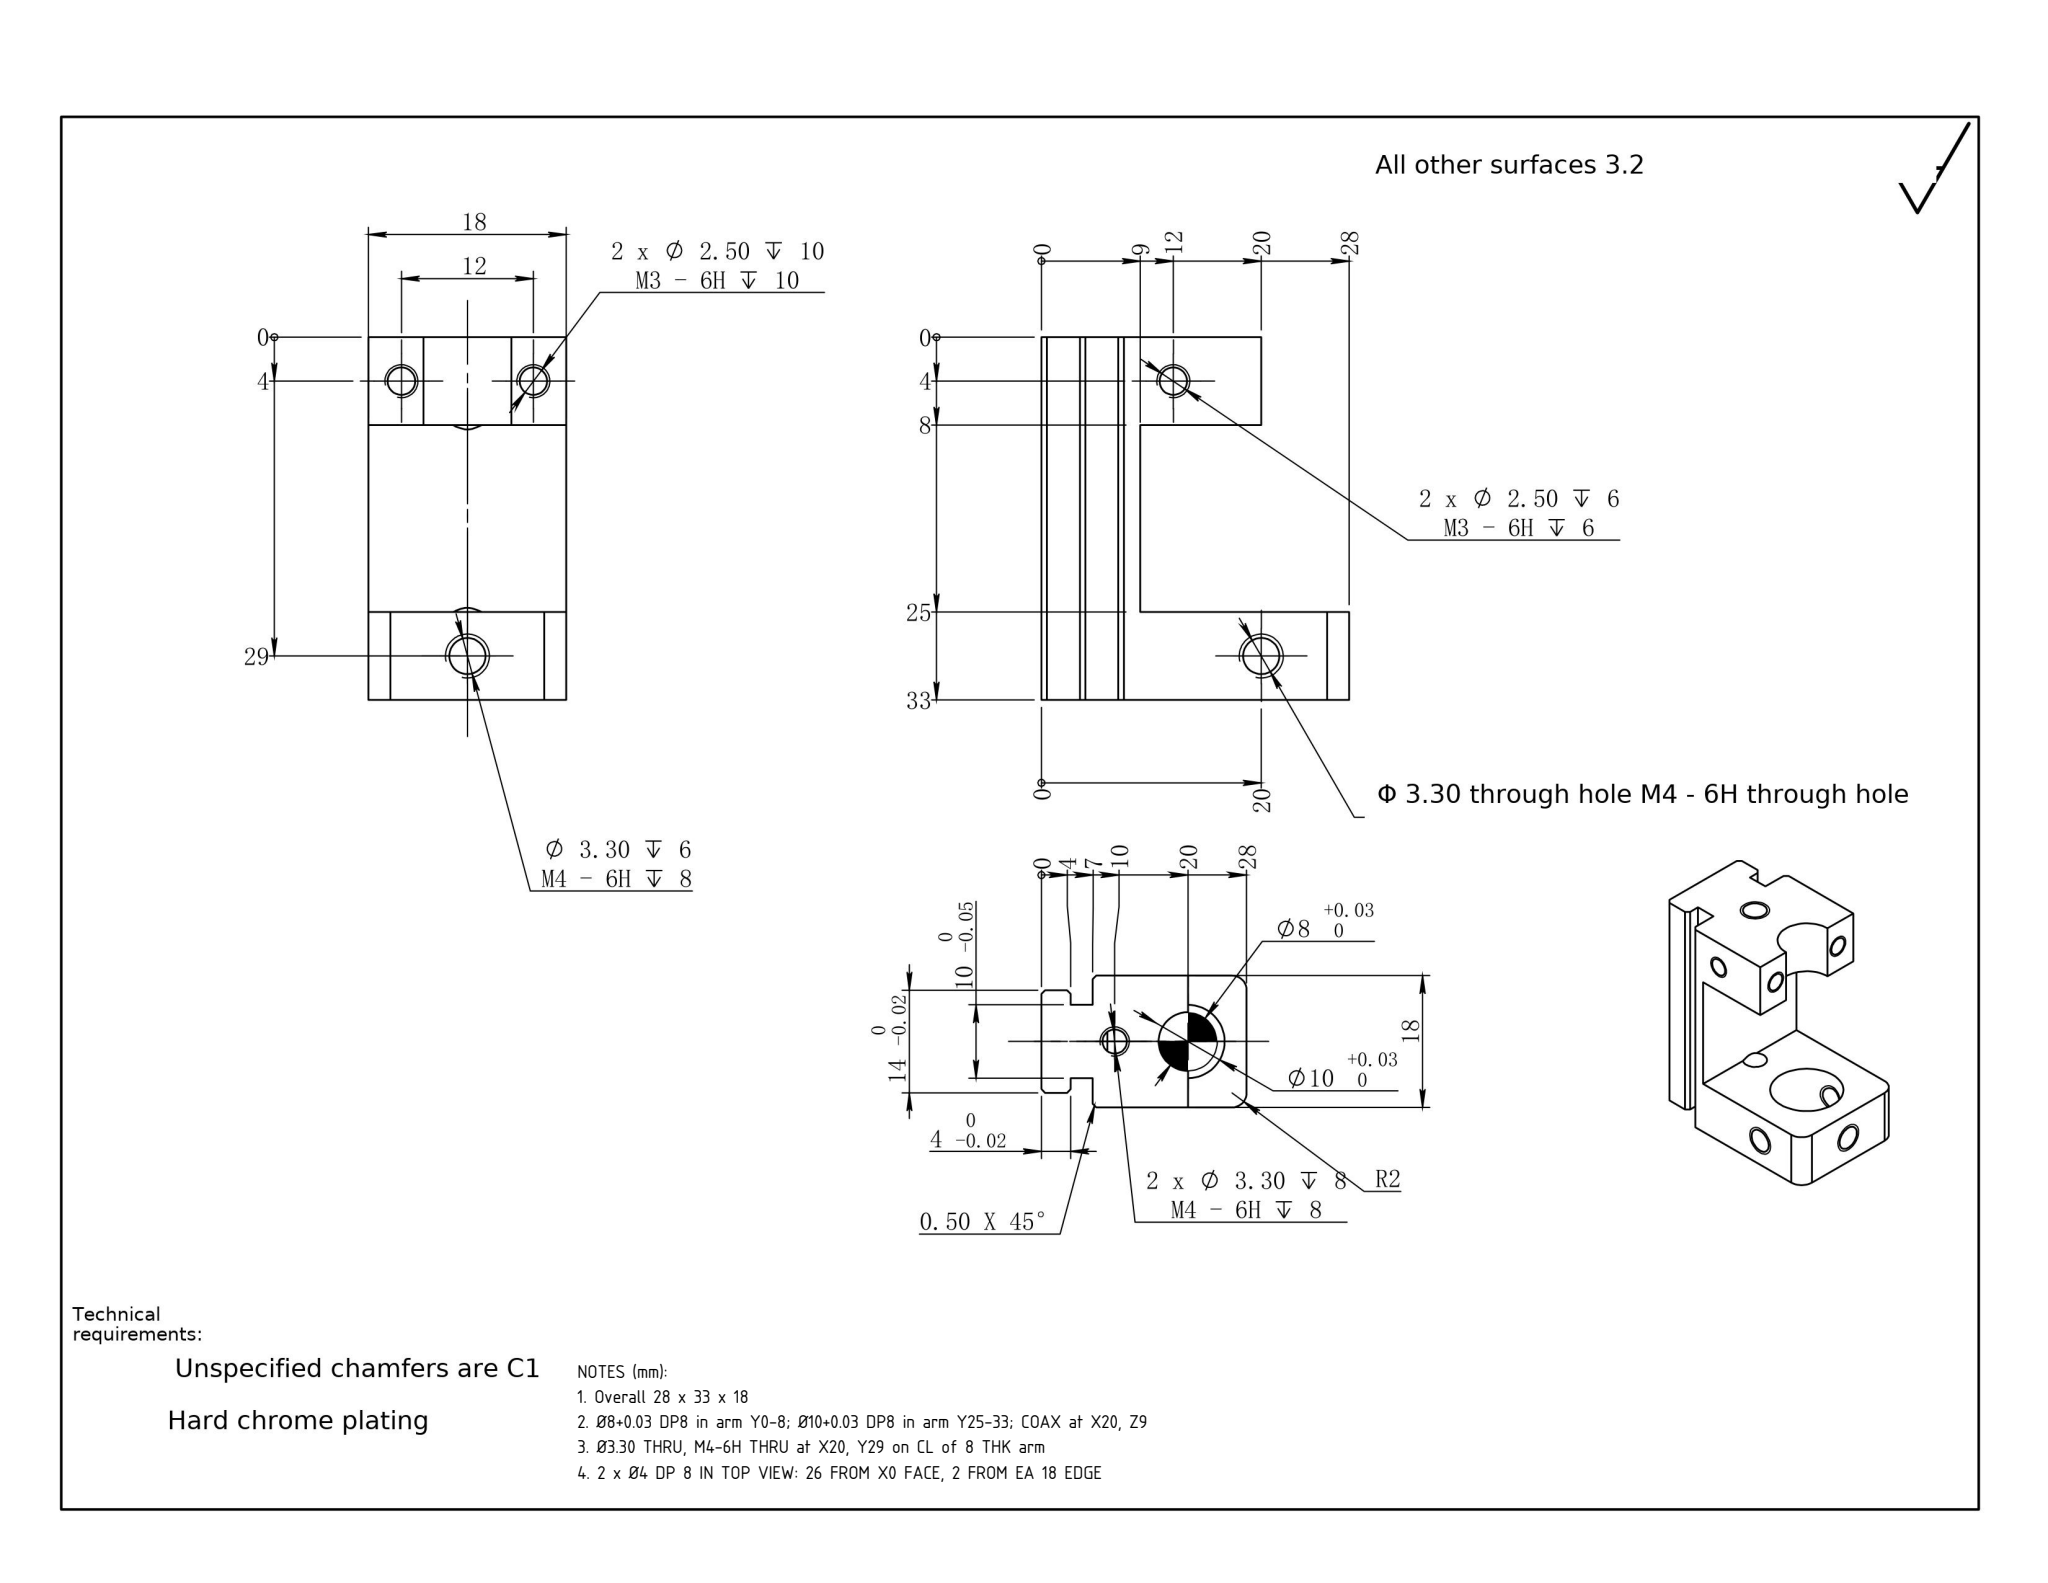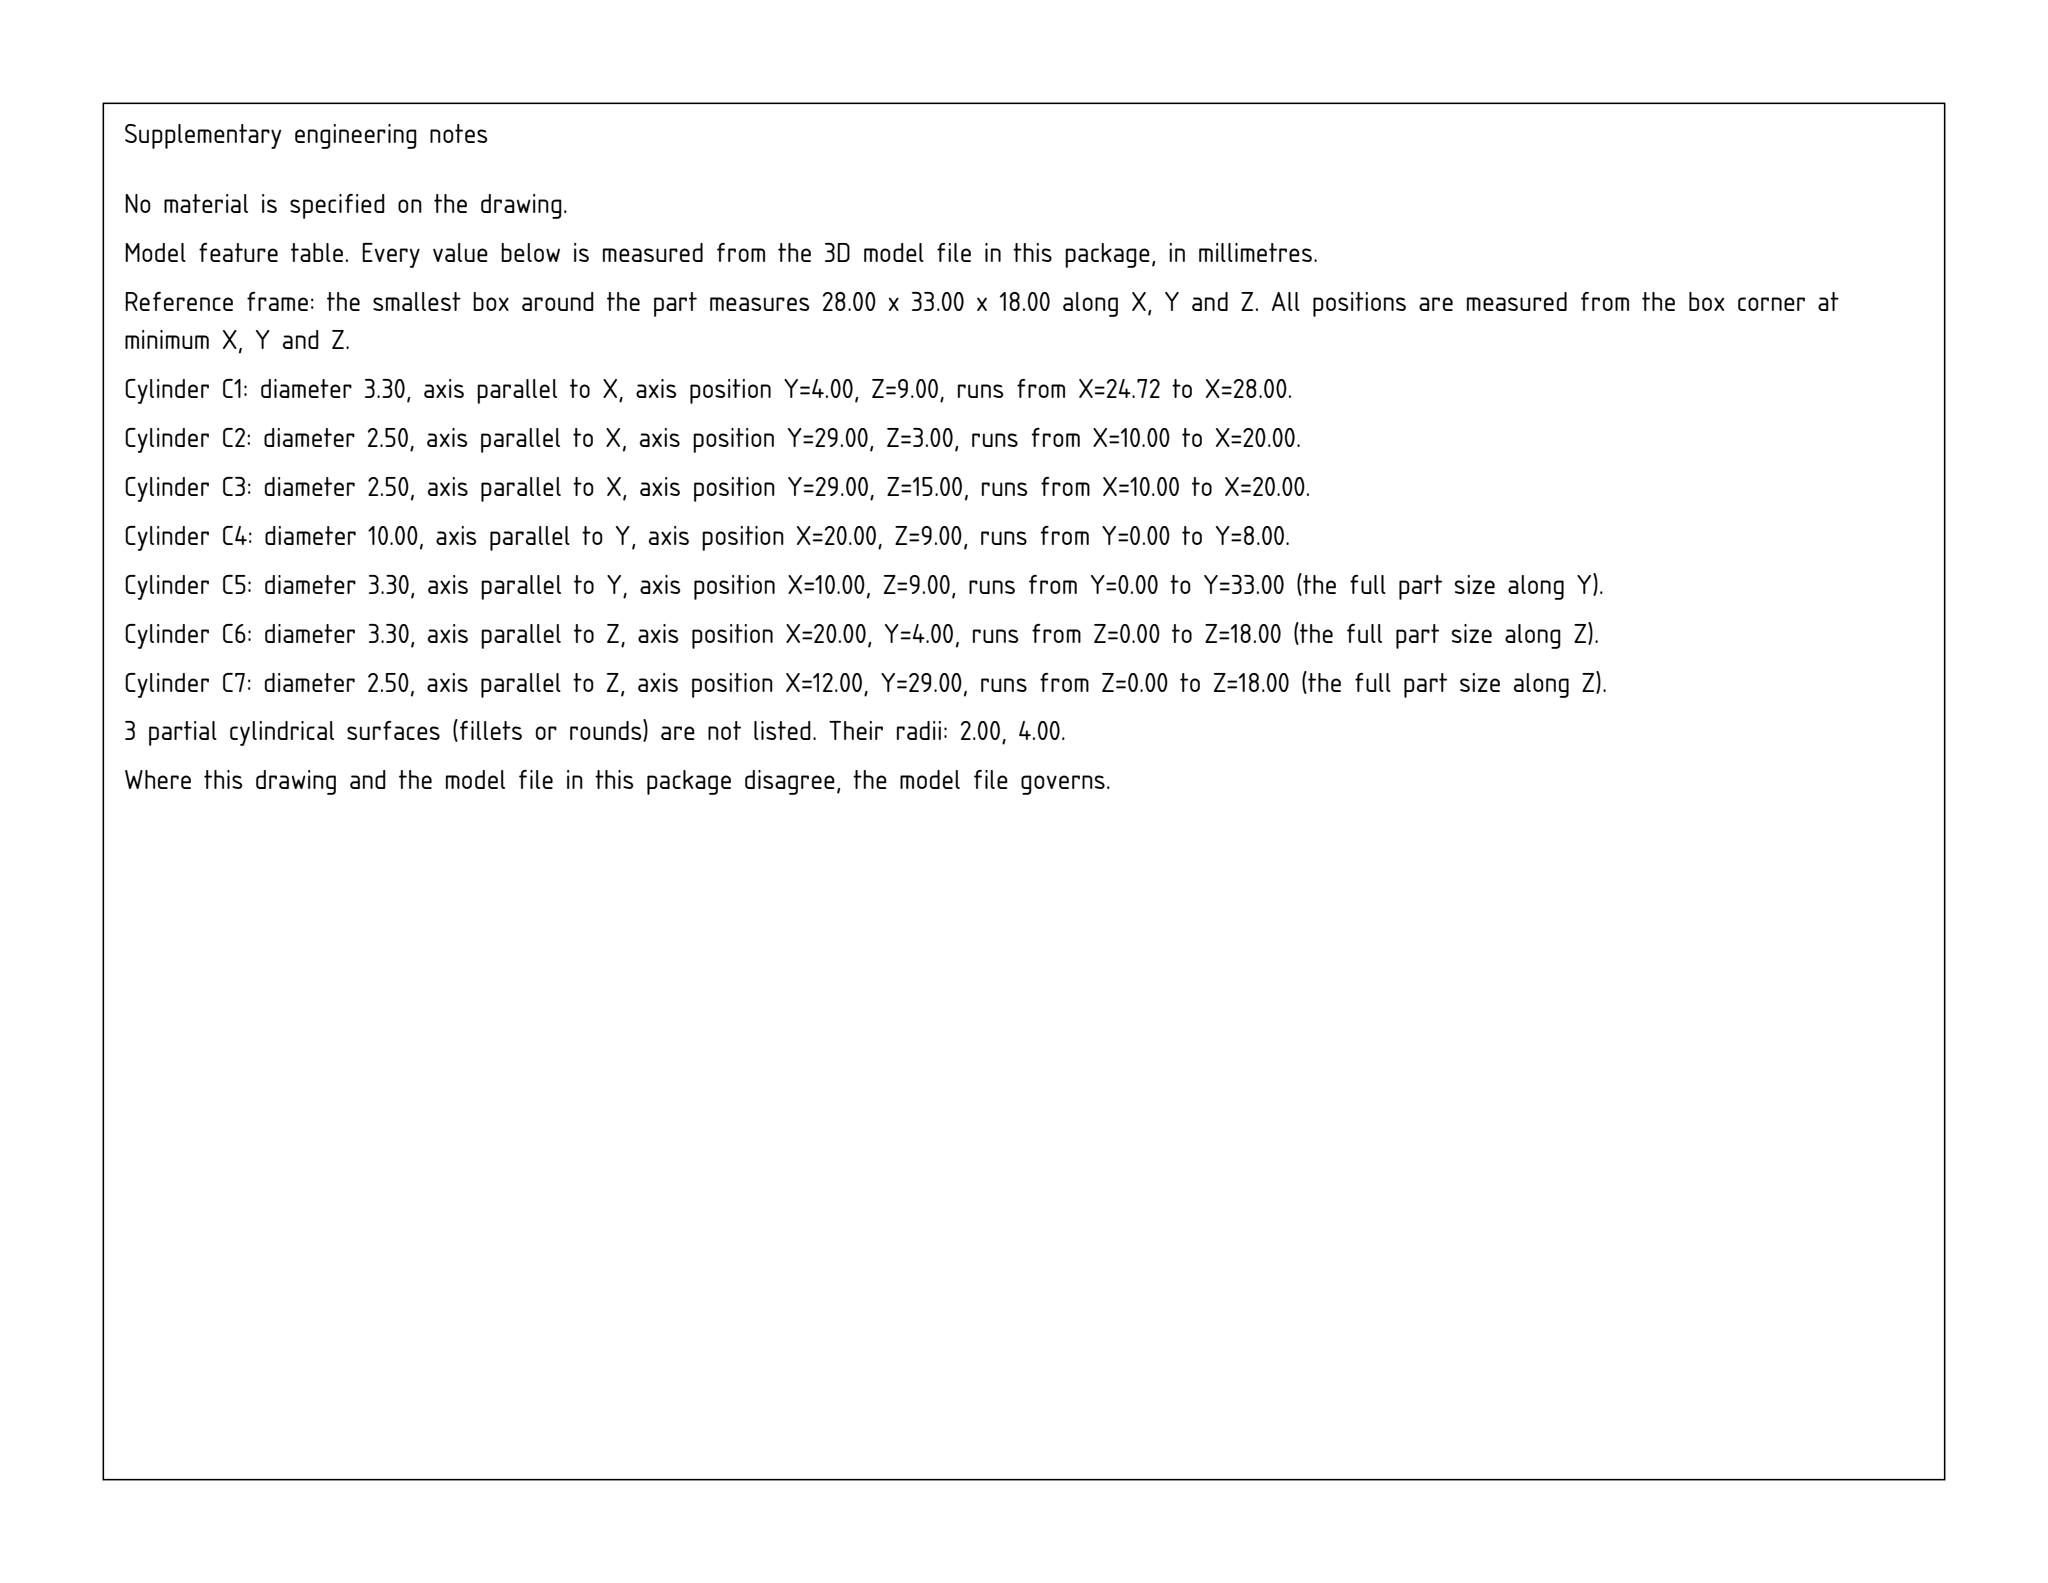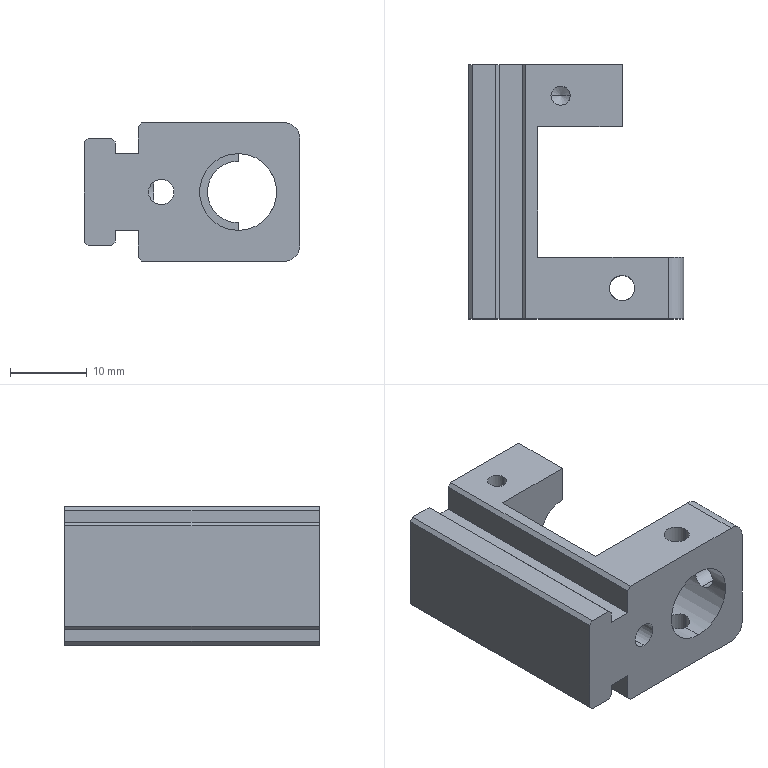Part | SolidWorks | mm | 1 solid | 66 faces | box 28 x 33 x 18 mm | volume 7104 mm3 | cylinder 31 | plane 25 | cone 10 | commonest cylinder face diameters 2.5 x16 3.3 x10 10 x2 4 x2 8 x1
Drawing notes:
Overall 28 x 33 x 18 | from the solid: bbox_xyz [28.001, 33.001, 18.001]
Ø8+0.03 DP8 in arm Y0-8; Ø10+0.03 DP8 in arm Y25-33; COAX at X20, Z9 | from the solid: cylinders [8.0,'y',[20,null,9],8.0] and [10.0,'y',[20,null,9],8.0]; arm faces y0/8 and y25/33 give 8 THK; Ø3.3 x-hole L3.28 and Ø3.3 z-hole L4.28 break into r5 bore, placing Ø10 in the M4-hole arm
Ø3.30 THRU, M4-6H THRU at X20, Y29 on CL of 8 THK arm | from the solid: cylinder [3.3,'z',[20,4(model),null],4.28] = drawing Y 33-4 = 29; arm faces y25/y33
2 x Ø4 DP 8 IN TOP VIEW: 26 FROM X0 FACE, 2 FROM EA 18 EDGE | from the solid: cylinders [4.0,"y",[26.0,null,2.0],8.0] and [4.0,"y",[26.0,null,16.0],8.0]; bbox 28 x 33 x 18, Z planes 0 and 18
build123d program:
from build123d import *

# Parameters (mm, degrees)
SKETCH2_W             = 18
SKETCH2_H             = 33
BOSS_EXTRUDE1_DEPTH   = 28
SKETCH3_W             = 38
SKETCH3_H             = 17
CUT_EXTRUDE1_DEPTH    = 38.152
SKETCH5_R             = 4
CUT_EXTRUDE2_DEPTH    = 45.204
SKETCH6_W             = 3
SKETCH6_H             = 8
CUT_EXTRUDE3_DEPTH    = 45.204
SKETCH14_W            = 4
SKETCH14_H            = 2
CUT_EXTRUDE5_DEPTH    = 45.204
SKETCH10_W            = 16
SKETCH10_H            = 18
CUT_EXTRUDE4_DEPTH    = 10
M3_TAPPED_HOLE1_D     = 2.5
M3_TAPPED_HOLE1_DEPTH = 10
M3_TAPPED_HOLE1_TIP   = 0.7511
CHAMFER1_SIZE         = 0.5
FILLET1_R             = 2
M4_TAPPED_HOLE2_D     = 3.3
M4_TAPPED_HOLE2_DEPTH = 6
M4_TAPPED_HOLE2_TIP   = 0.9914
M4_TAPPED_HOLE3_D     = 3.3
SKETCH22_R            = 5
CUT_EXTRUDE6_DEPTH    = 10


with BuildPart() as part:
    # Sketch2 → Boss-Extrude1 (new body)
    with BuildSketch(Plane(origin=(0, 0, 0), x_dir=(0, 0, -1), z_dir=(1, 0, 0))):
        Rectangle(SKETCH2_W, SKETCH2_H)
    extrude(amount=BOSS_EXTRUDE1_DEPTH)

    # Sketch3 → Cut-Extrude1 (cut, through all)
    with BuildSketch(Plane.XY.offset(9)):
        with Locations((28, 0)):
            Rectangle(SKETCH3_W, SKETCH3_H)
    extrude(amount=-CUT_EXTRUDE1_DEPTH, mode=Mode.SUBTRACT)

    # Sketch5 → Cut-Extrude2 (cut, through all)
    with BuildSketch(Plane(origin=(0, 16.5, 0), x_dir=(1, 0, 0), z_dir=(0, 1, 0))):
        with Locations(Location((20, 0, 0), (0, 0, 270))):
            Circle(SKETCH5_R)
    extrude(amount=-CUT_EXTRUDE2_DEPTH, mode=Mode.SUBTRACT)

    # Sketch6 → Cut-Extrude3 (cut, through all)
    with BuildSketch(Plane(origin=(0, 16.5, 0), x_dir=(1, 0, 0), z_dir=(0, 1, 0))):
        with Locations((5.5, 9)):
            Rectangle(SKETCH6_W, SKETCH6_H)
        with Locations((5.5, -9)):
            Rectangle(SKETCH6_W, SKETCH6_H)
    extrude(amount=-CUT_EXTRUDE3_DEPTH, mode=Mode.SUBTRACT)

    # Sketch14 → Cut-Extrude5 (cut, through all)
    with BuildSketch(Plane(origin=(0, 16.5, 0), x_dir=(1, 0, 0), z_dir=(0, 1, 0))):
        with Locations((2, 8)):
            Rectangle(SKETCH14_W, SKETCH14_H)
        with Locations((2, -8)):
            Rectangle(SKETCH14_W, SKETCH14_H)
    extrude(amount=-CUT_EXTRUDE5_DEPTH, mode=Mode.SUBTRACT)

    # Sketch9 → M4 Tapped Hole1 (revolve, cut)
    with BuildSketch(Plane(origin=(10, 16.5, 0), x_dir=(0, 0, 1), z_dir=(1, 0, 0))):
        Polygon((0, 0), (0, 8.991), (1.65, 8), (1.65, 0), align=None)
    m4_tapped_hole1 = revolve(axis=Axis((10, 22.85, 0), (0, -1, 0)), mode=Mode.SUBTRACT)

    # Sketch10 → Cut-Extrude4 (cut)
    with BuildSketch(Plane(origin=(0, 16.5, 0), x_dir=(1, 0, 0), z_dir=(0, 1, 0))):
        with Locations((28, 0)):
            Rectangle(SKETCH10_W, SKETCH10_H)
    extrude(amount=-CUT_EXTRUDE4_DEPTH, mode=Mode.SUBTRACT)

    # M3 Tapped Hole1
    with Locations(Plane(origin=(20, 0, 0), x_dir=(0, 0, -1), z_dir=(1, 0, 0))):
        with Locations((-6, 12.5), (6, 12.5)):
            Hole(M3_TAPPED_HOLE1_D / 2, depth=M3_TAPPED_HOLE1_DEPTH)
            with Locations((0, 0, -(M3_TAPPED_HOLE1_DEPTH + M3_TAPPED_HOLE1_TIP / 2))):  # 118° drill point
                Cone(0, M3_TAPPED_HOLE1_D / 2, M3_TAPPED_HOLE1_TIP, mode=Mode.SUBTRACT)

    # Chamfer1
    chamfer1_edges = [part.edges().sort_by_distance(p)[0] for p in [
        (7, 0, -9),
        (7, 0, 9),
        (4, 0, -7),
        (0, 0, -7),
        (4, 0, 7),
        (0, 0, 7),
    ]]
    chamfer(chamfer1_edges, length=CHAMFER1_SIZE)

    # Fillet1
    fillet1_edges = [part.edges().sort_by_distance(p)[0] for p in [
        (28, -12.5, 9),
        (28, -12.5, -9),
    ]]
    fillet(fillet1_edges, radius=FILLET1_R)

    # Sketch16 → M3 Tapped Hole2 (revolve, cut)
    with BuildSketch(Plane(origin=(12, 12.5, 9), x_dir=(0, -1, 0), z_dir=(1, 0, 0))):
        Polygon((0, 0), (0, 6.751), (1.25, 6), (1.25, 0), align=None)
    m3_tapped_hole2 = revolve(axis=Axis((12, 12.5, 15.35), (0, 0, -1)), mode=Mode.SUBTRACT)

    # Mirror1: M3 Tapped Hole2 across plane
    add(m3_tapped_hole2.mirror(Plane.XY), mode=Mode.SUBTRACT)

    # M4 Tapped Hole2
    with Locations(Plane(origin=(28, 0, 0), x_dir=(0, 0, -1), z_dir=(1, 0, 0))):
        with Locations((0, -12.5)):
            Hole(M4_TAPPED_HOLE2_D / 2, depth=M4_TAPPED_HOLE2_DEPTH)
            with Locations((0, 0, -(M4_TAPPED_HOLE2_DEPTH + M4_TAPPED_HOLE2_TIP / 2))):  # 118° drill point
                Cone(0, M4_TAPPED_HOLE2_D / 2, M4_TAPPED_HOLE2_TIP, mode=Mode.SUBTRACT)

    # M4 Tapped Hole3 (through all)
    with Locations(Plane.XY.offset(9)):
        with Locations((20, -12.5)):
            Hole(M4_TAPPED_HOLE3_D / 2)

    # Mirror2: M4 Tapped Hole1 across plane
    add(m4_tapped_hole1.mirror(Plane.ZX), mode=Mode.SUBTRACT)

    # Sketch22 → Cut-Extrude6 (cut)
    with BuildSketch(Plane.XZ.offset(16.5)):
        with Locations(Location((20, 0, 0), (0, 0, 270))):
            Circle(SKETCH22_R)
    extrude(amount=-CUT_EXTRUDE6_DEPTH, mode=Mode.SUBTRACT)


solid = part.part